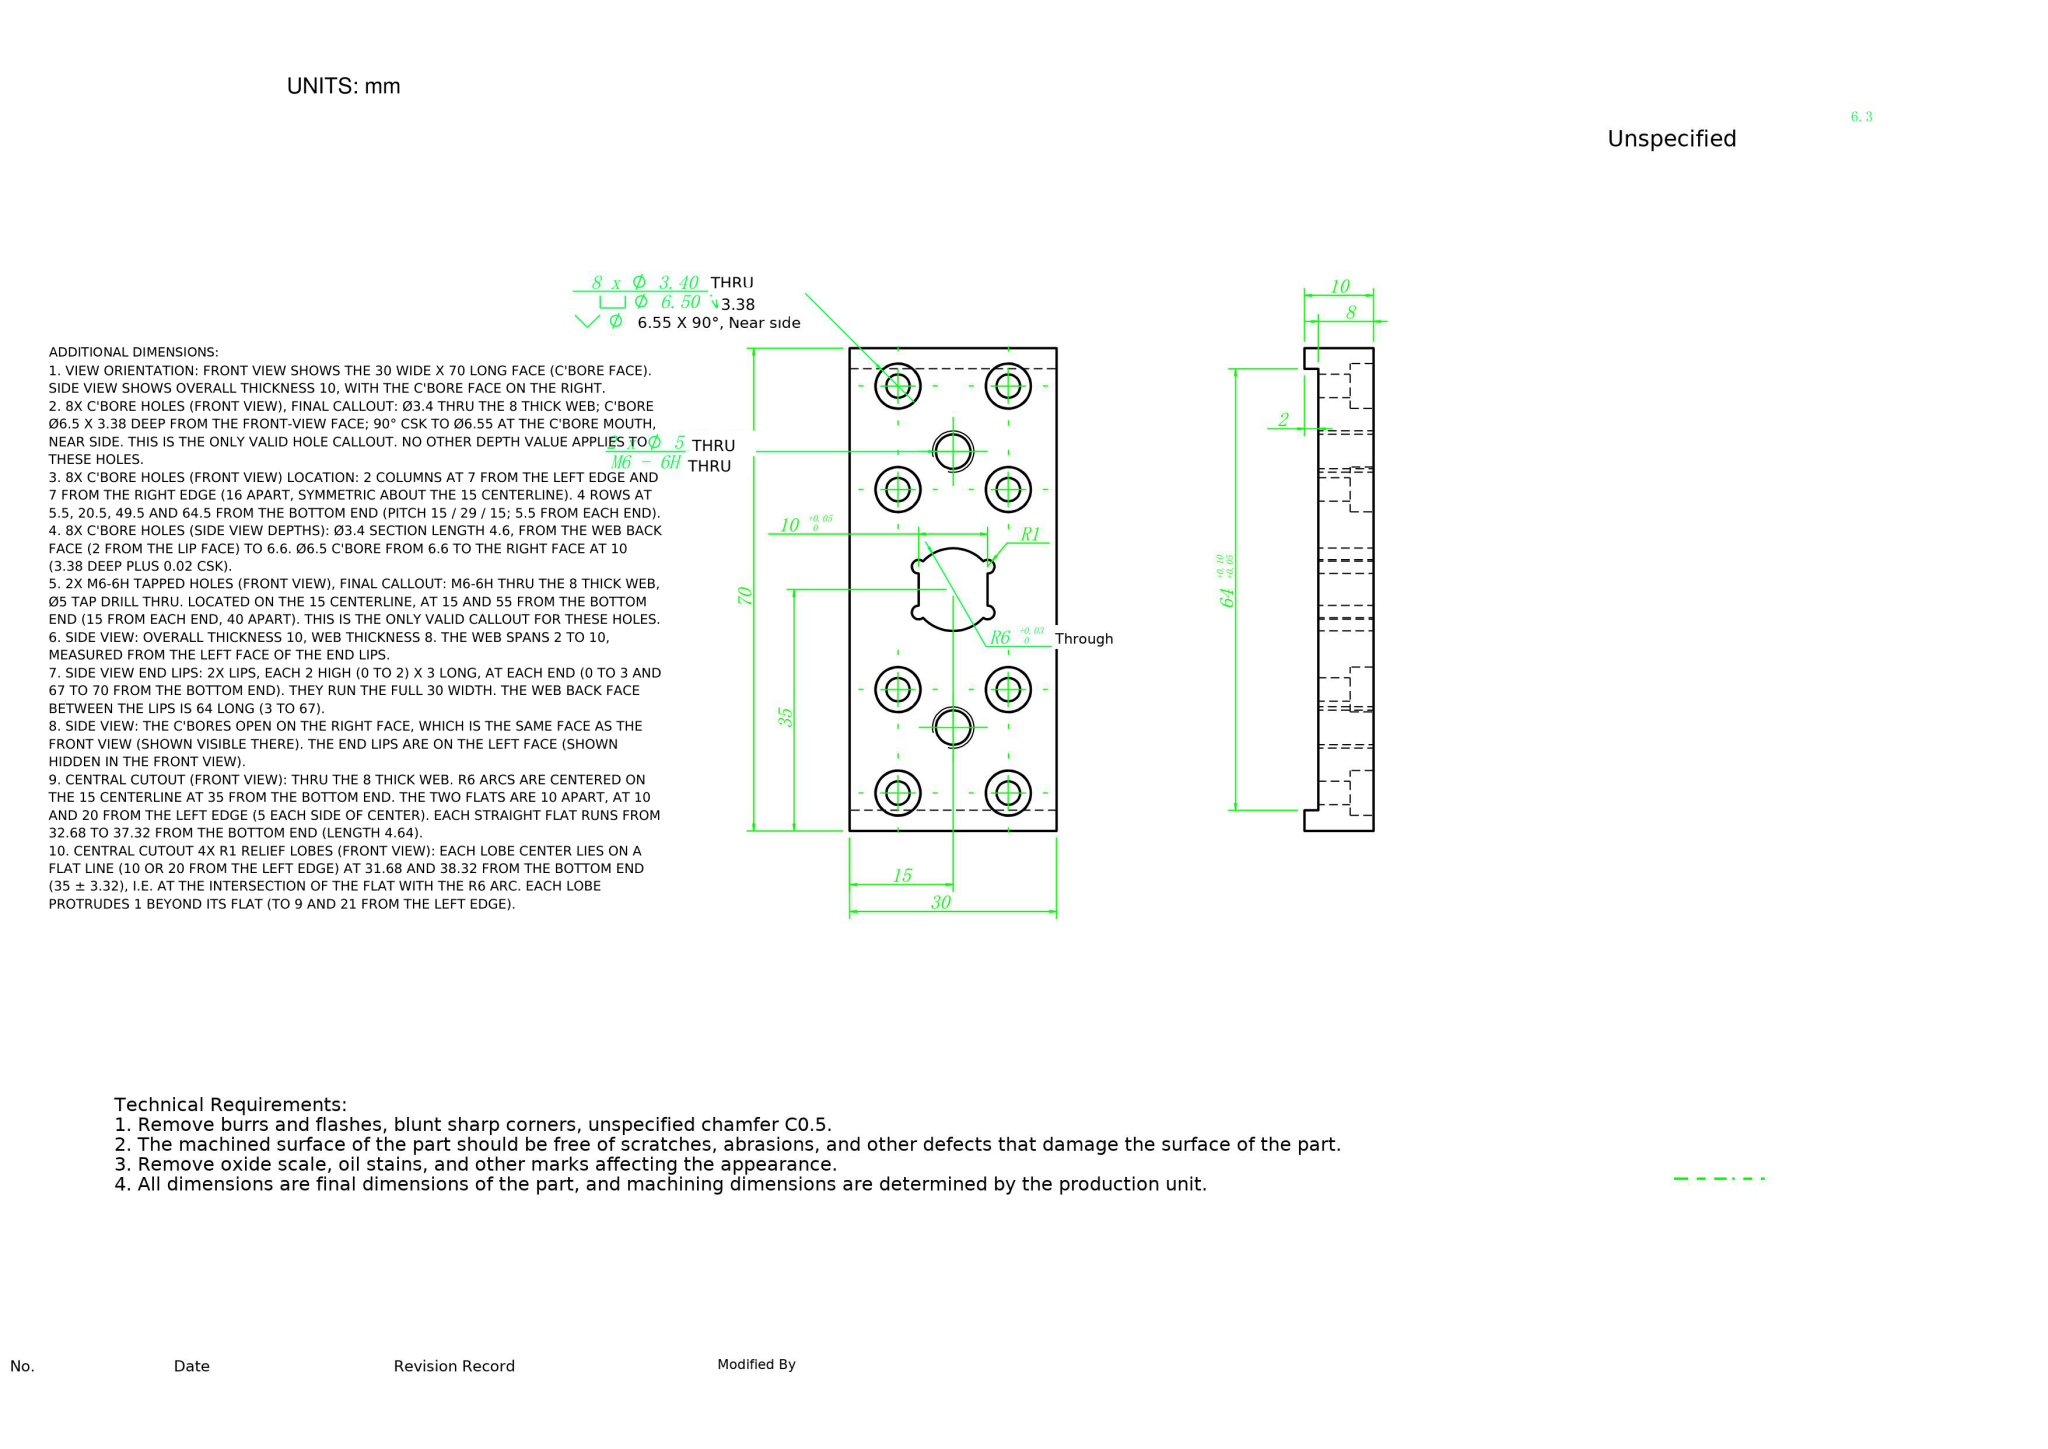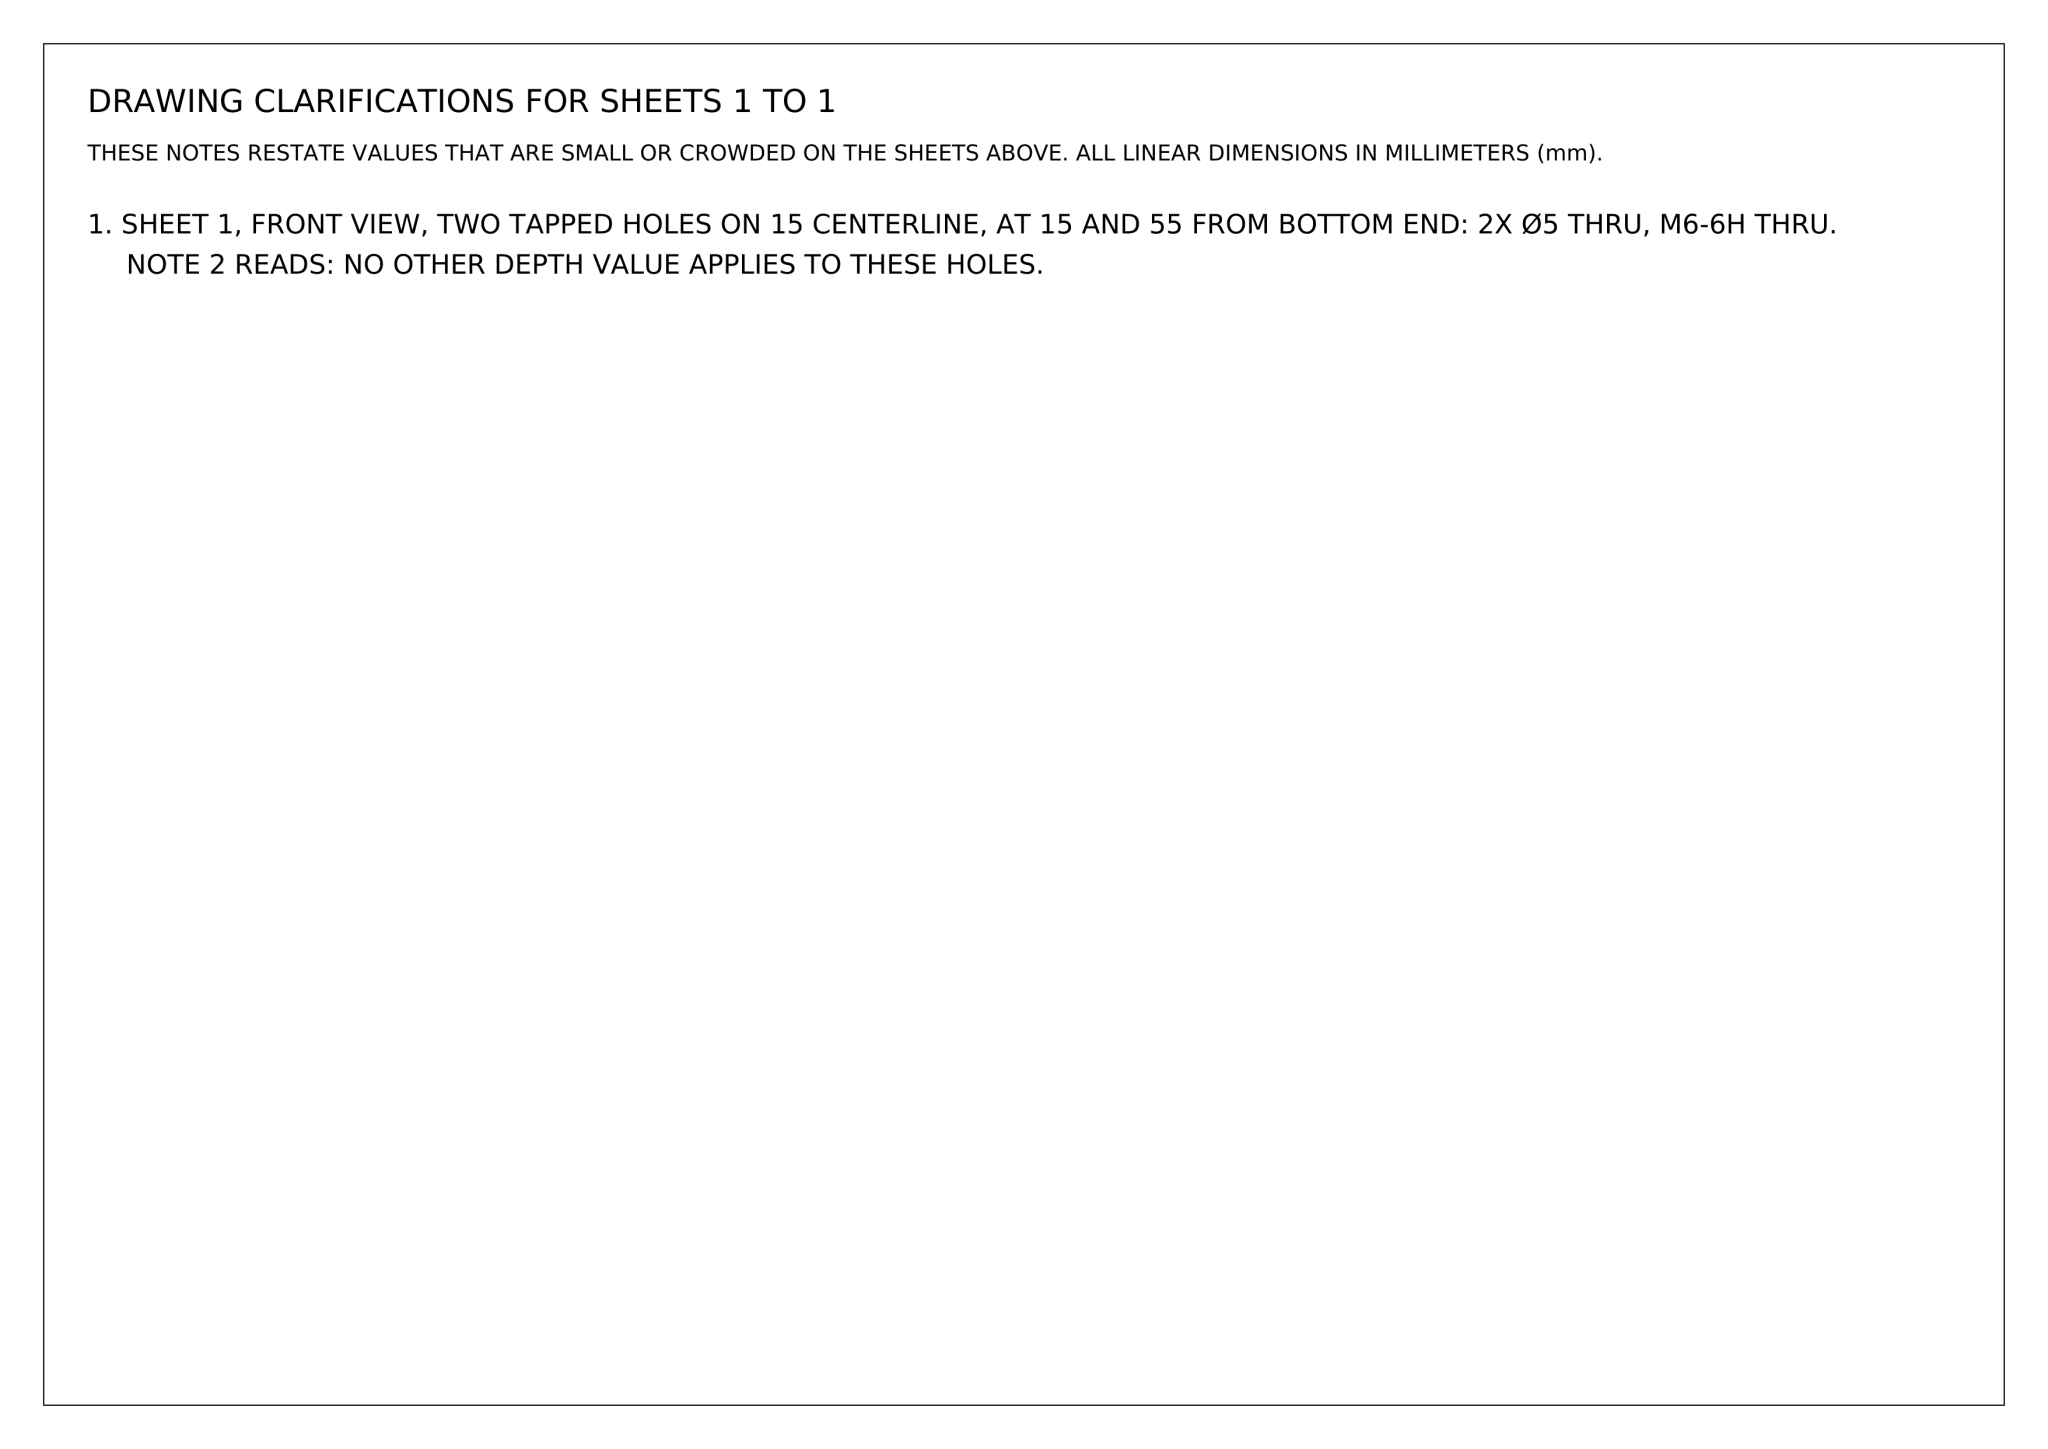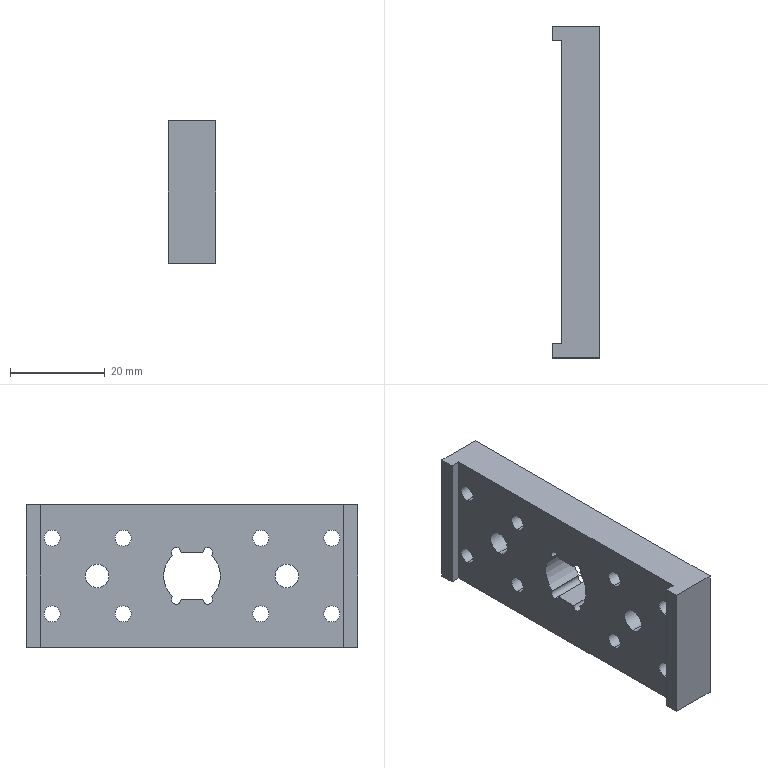Part | NX | mm | 1 solid | 80 faces | box 10 x 70 x 30 mm | volume 14716 mm3 | cylinder 44 | plane 20 | cone 16 | commonest cylinder face diameters 6.5 x16 3.4 x16 2 x6 5 x4 12 x2